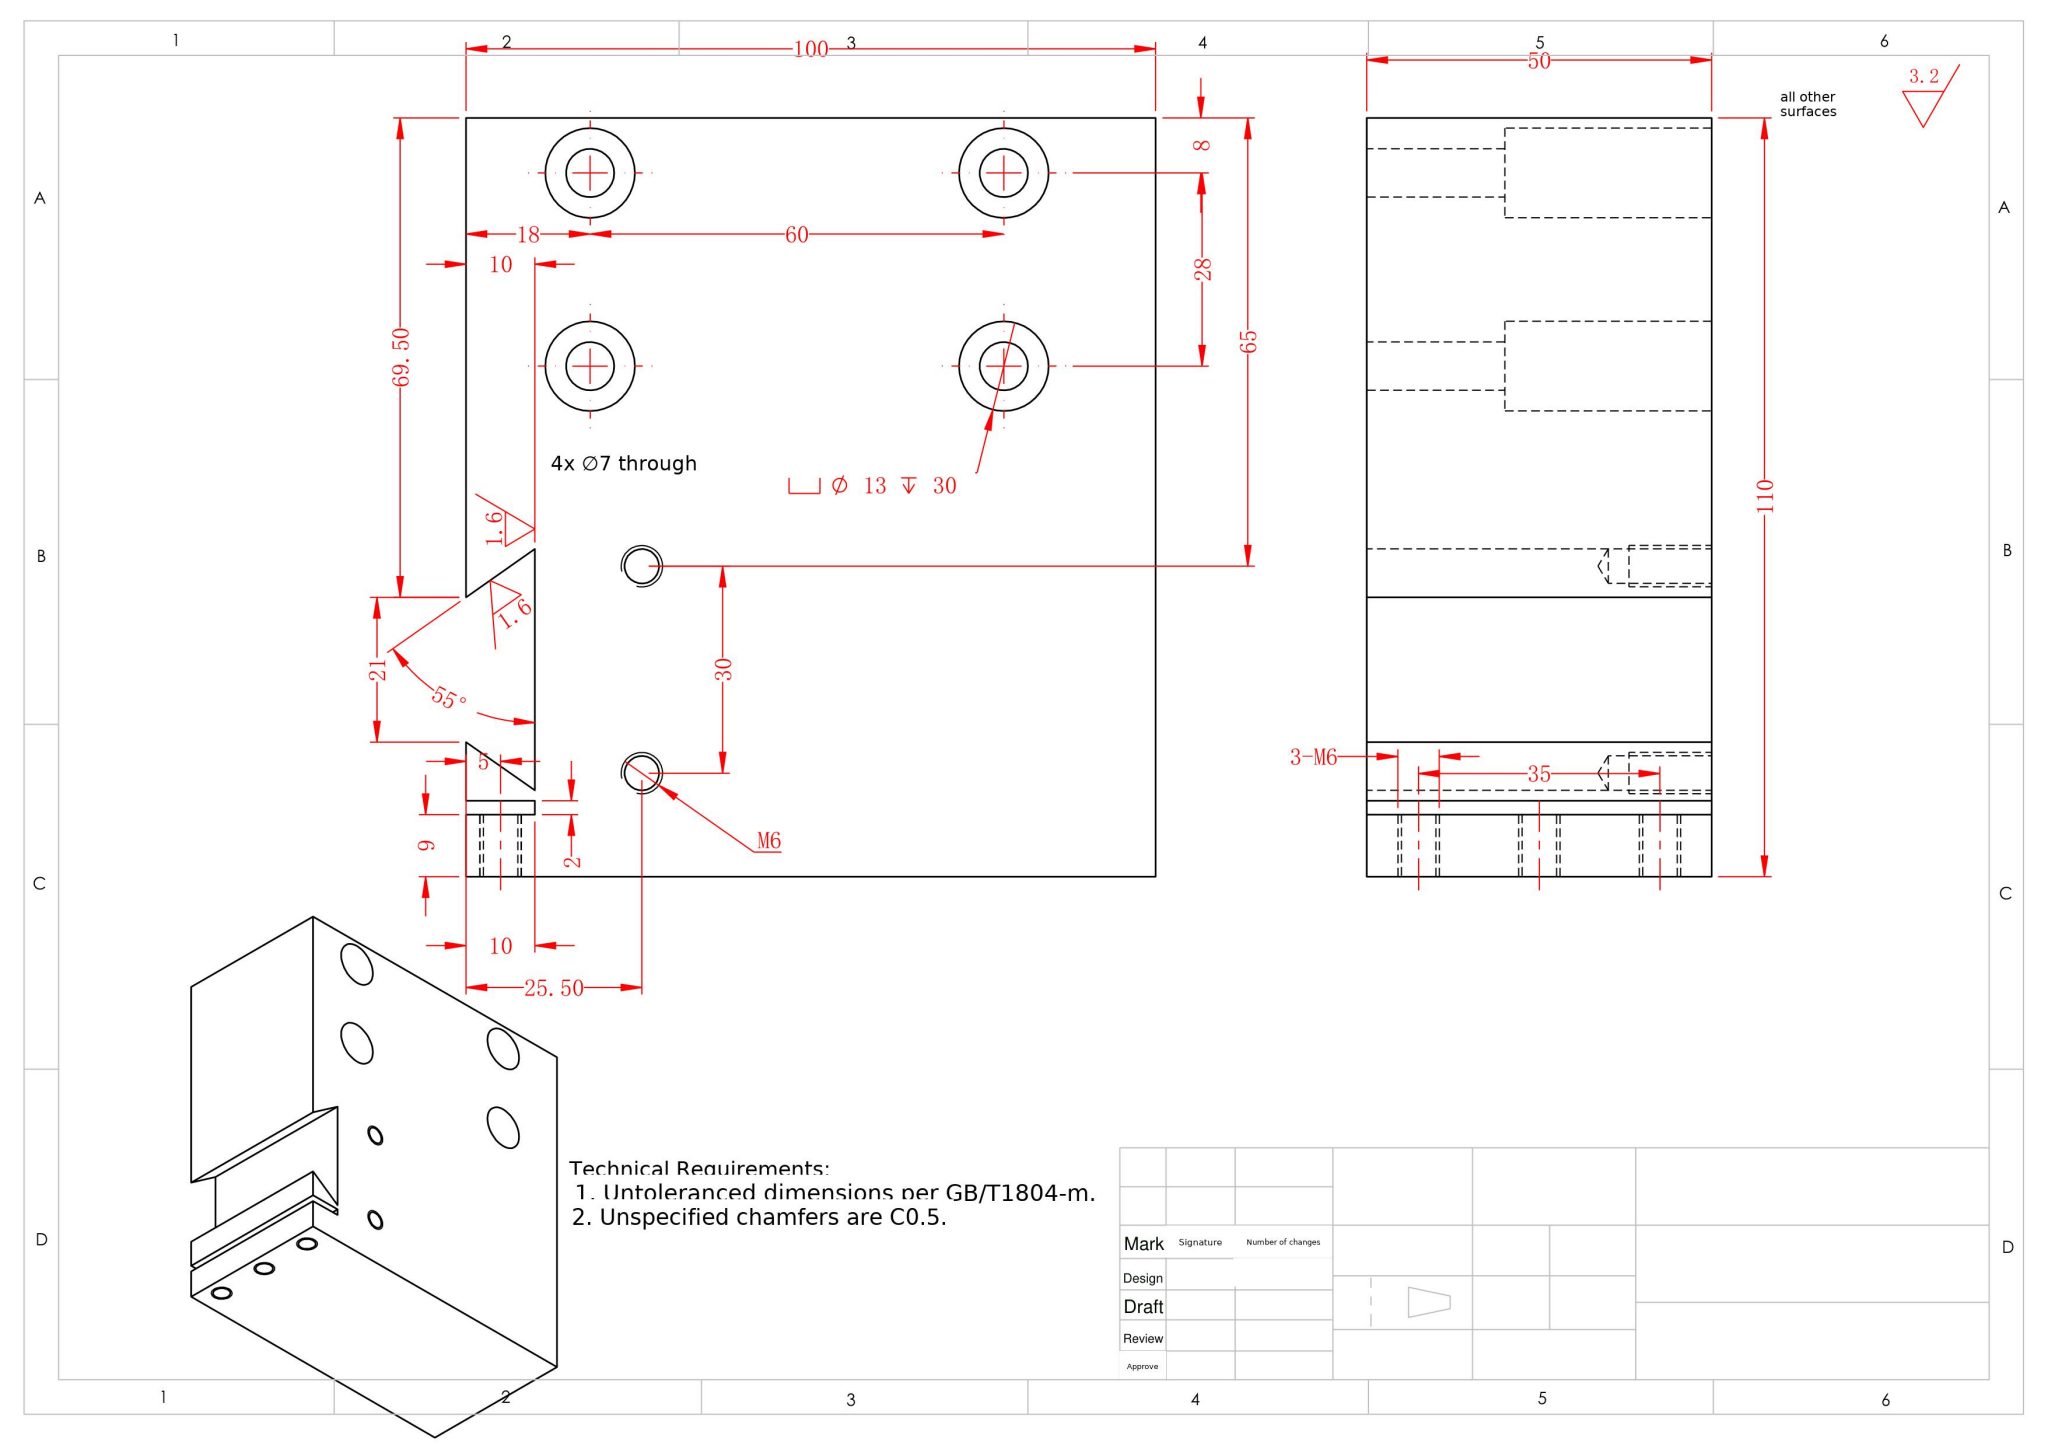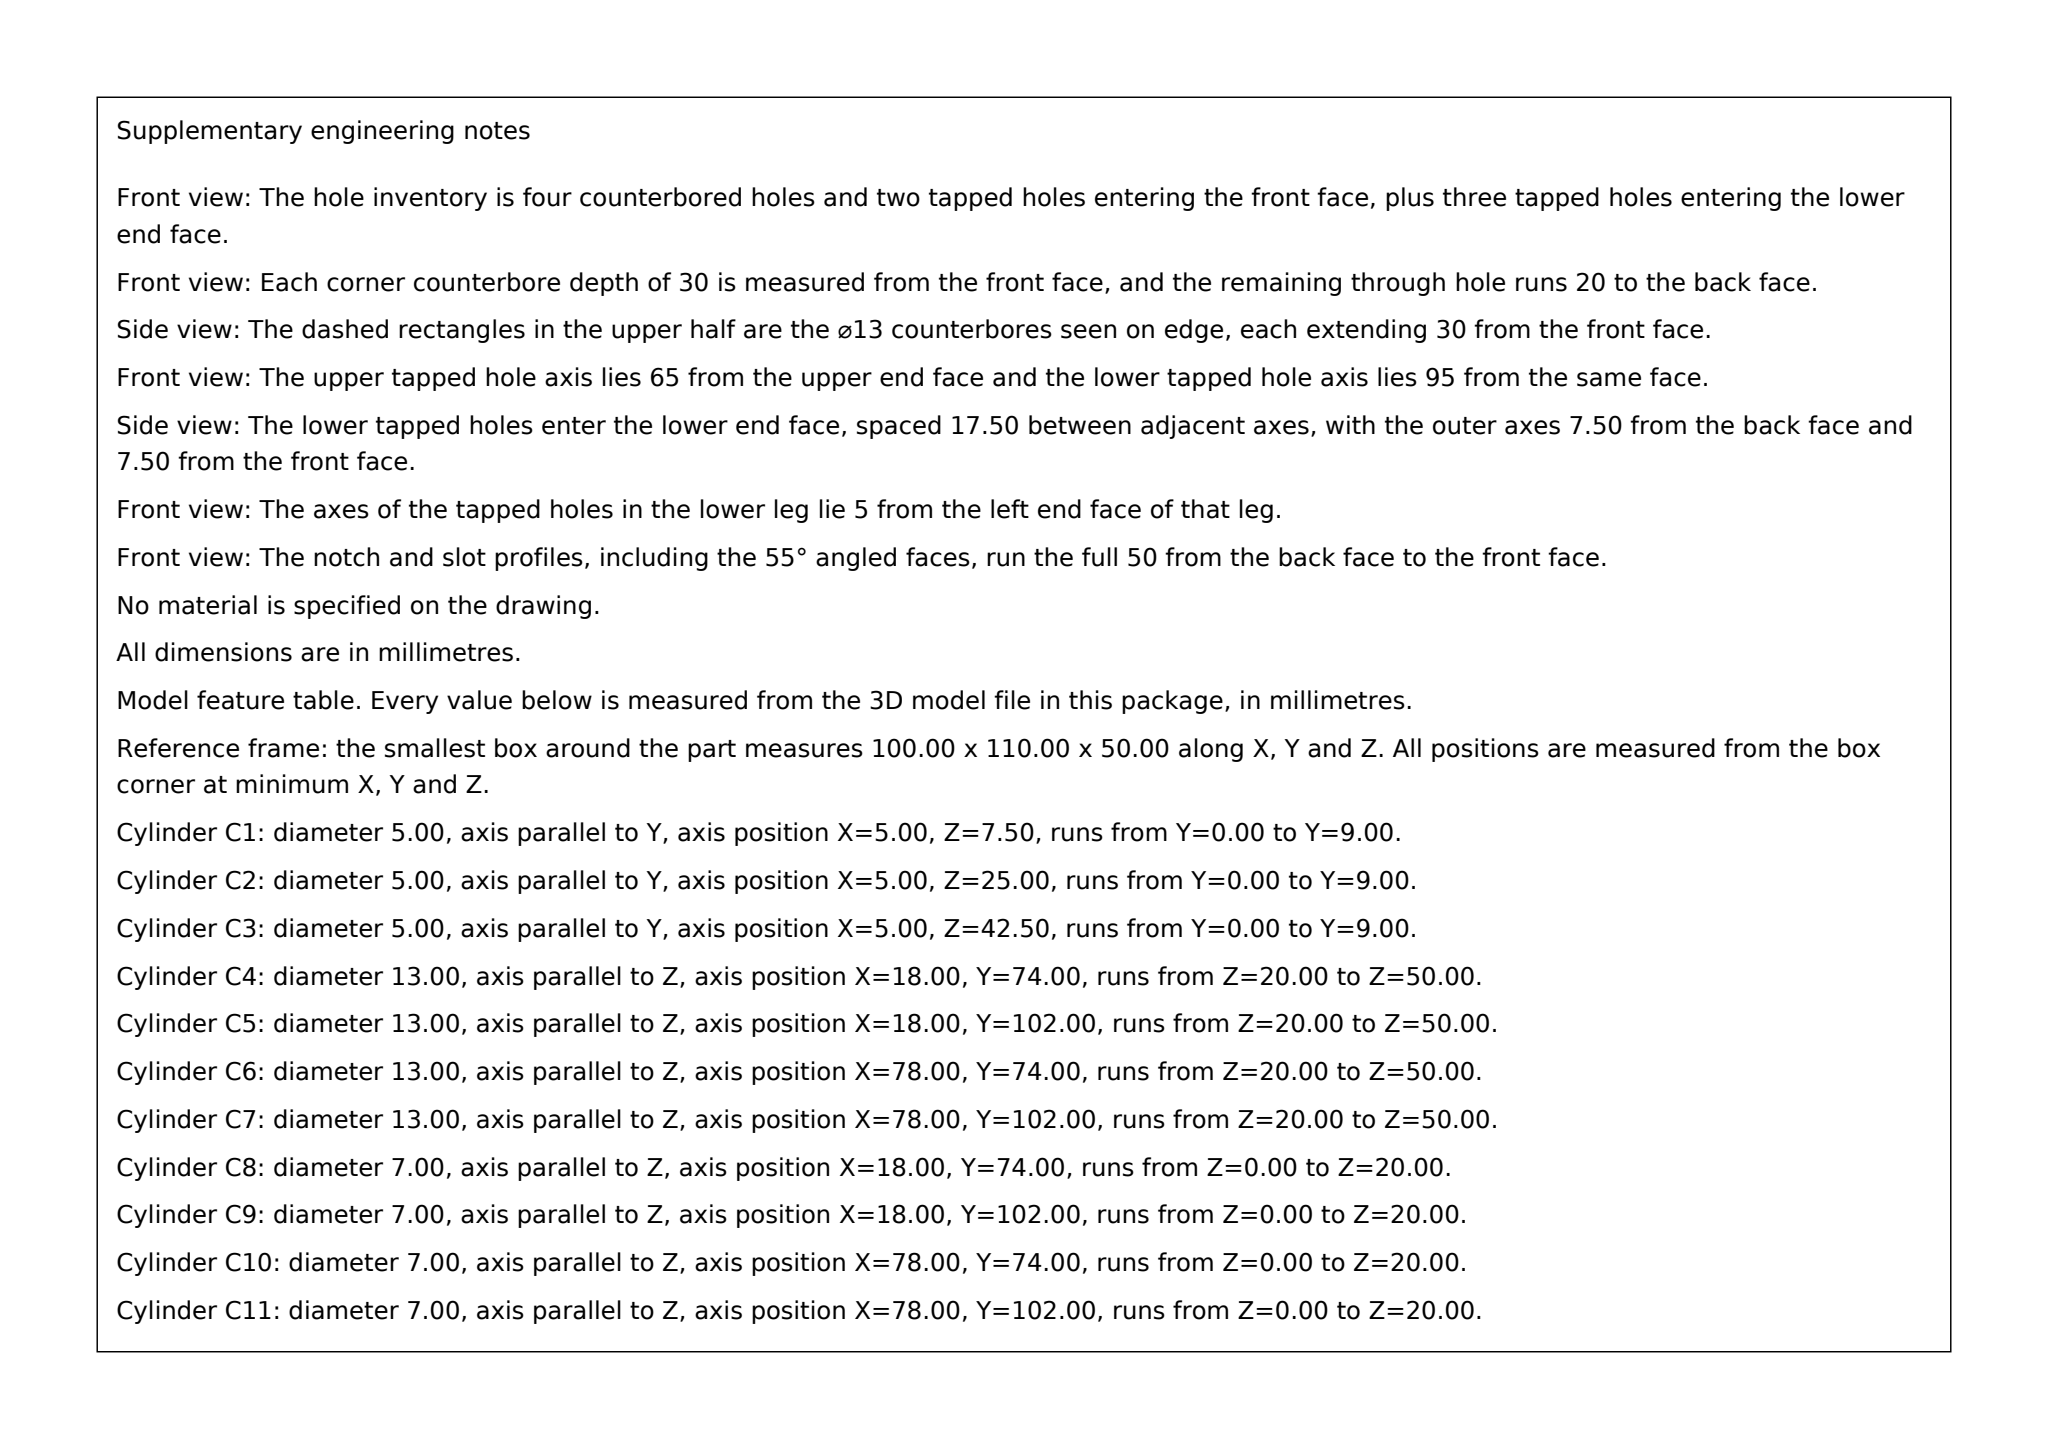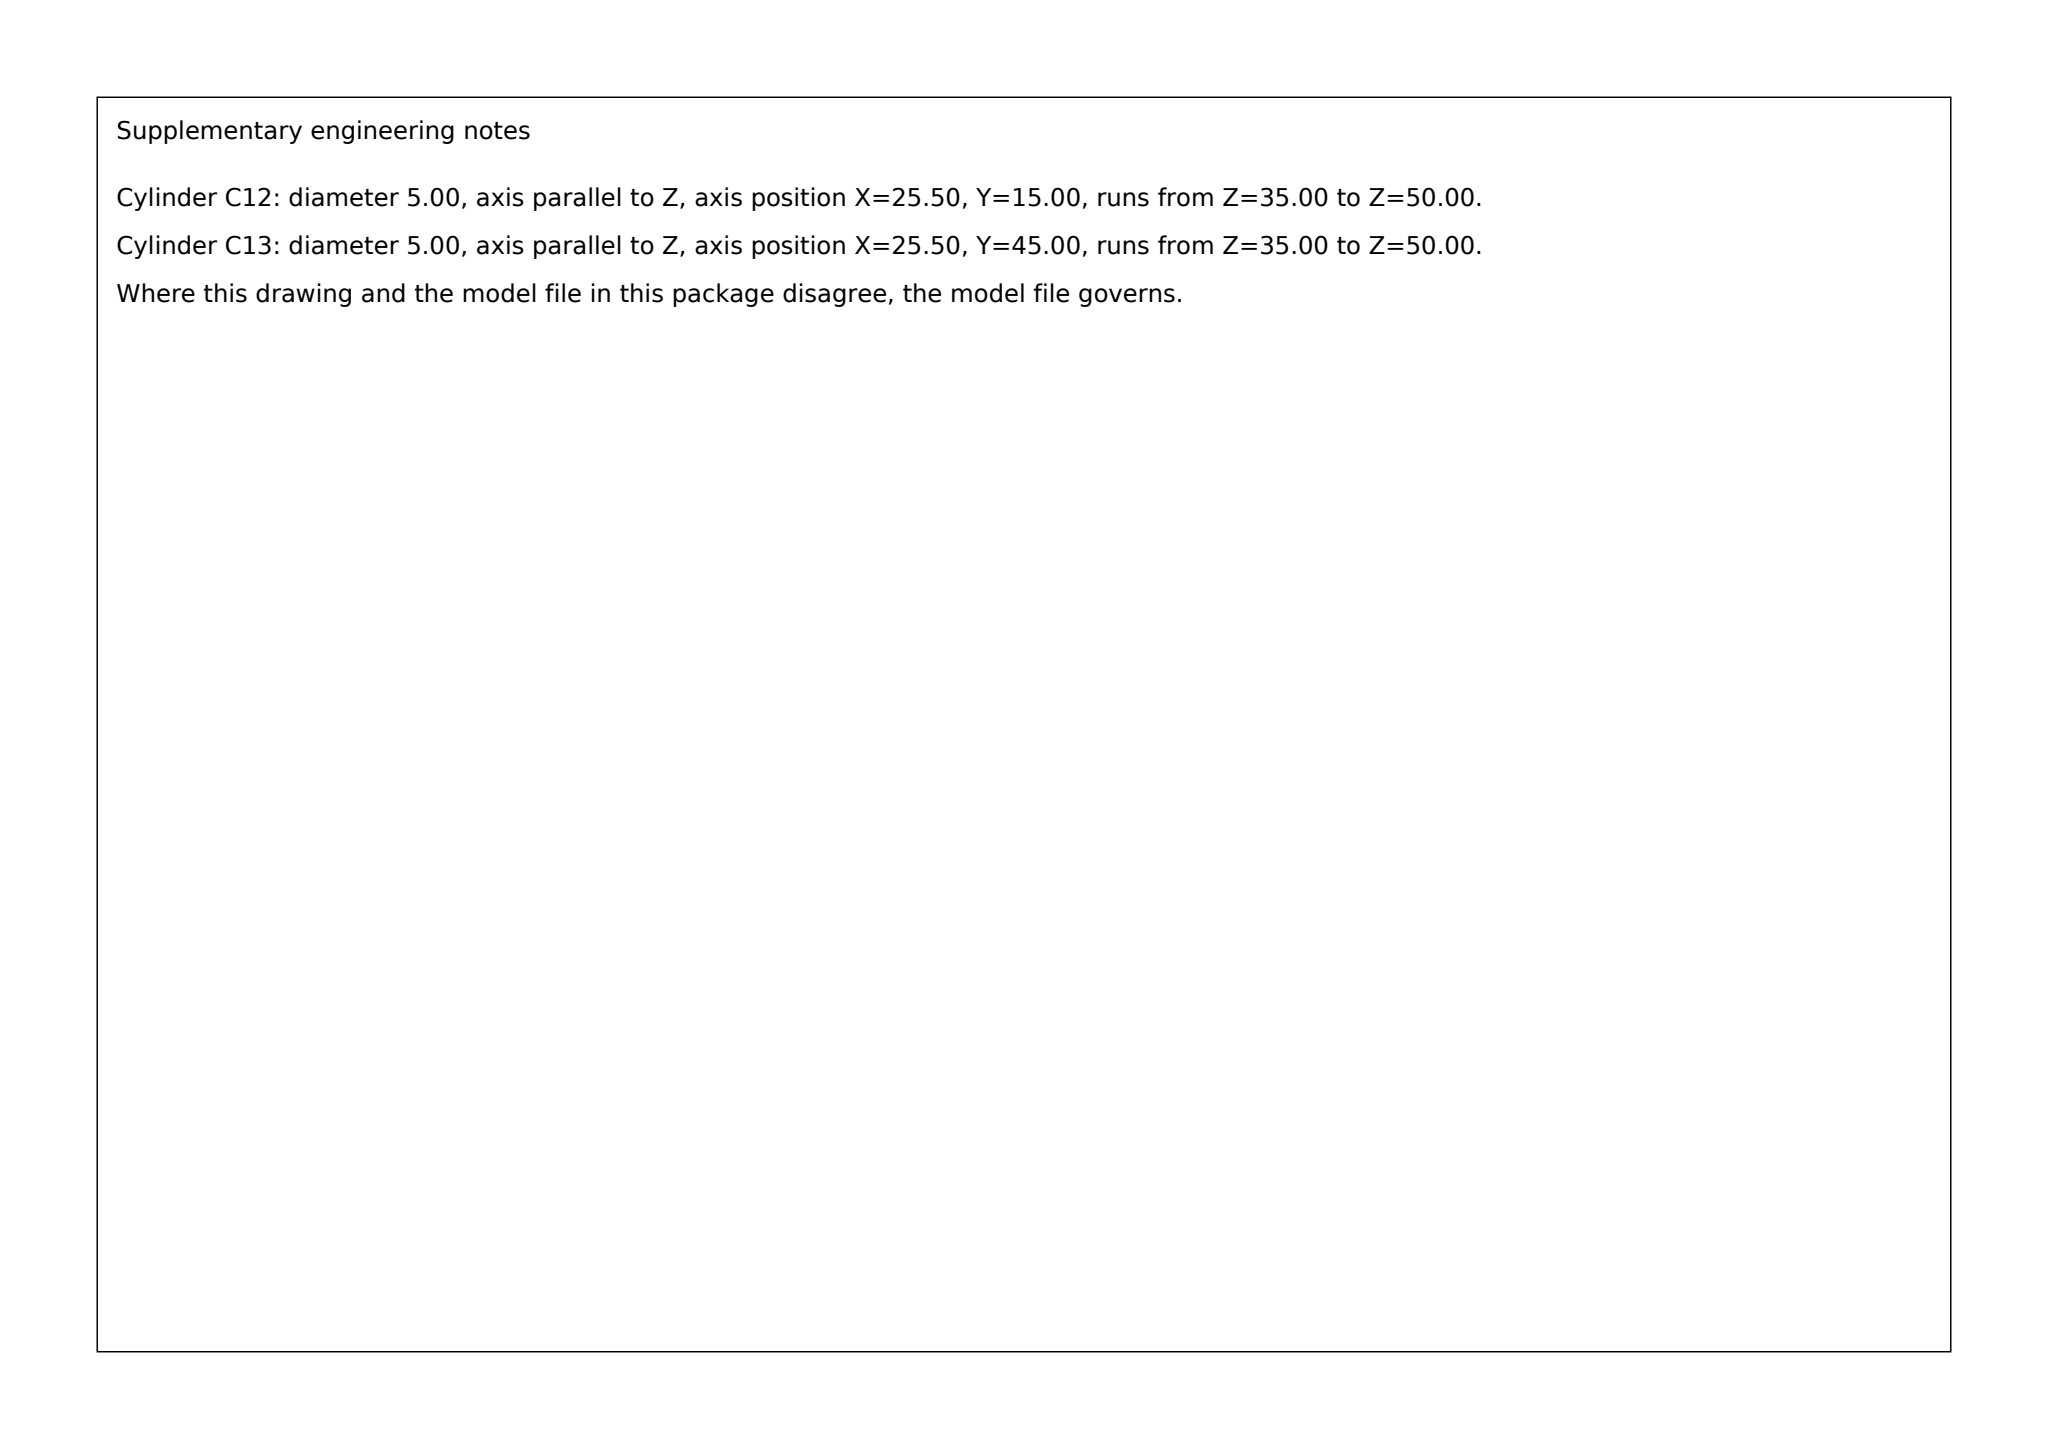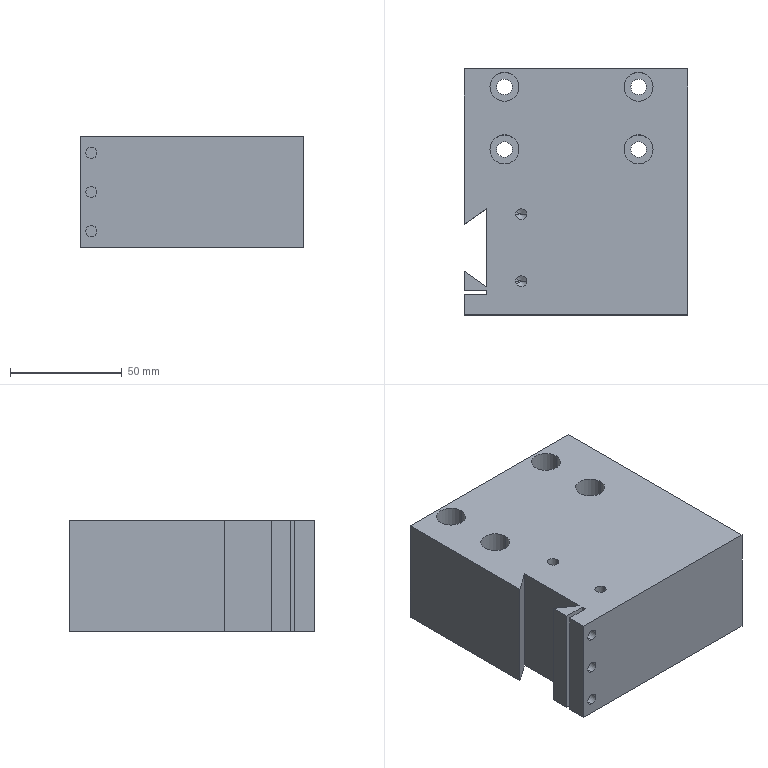Part | SolidWorks | mm | 1 solid | 48 faces | box 100 x 110 x 50 mm | volume 514856 mm3 | cylinder 26 | plane 18 | cone 4 | commonest cylinder face diameters 5 x10 13 x8 7 x8
Drawing notes:
3X M6 DP 9 IN FOOT: HOLE CL 5 FROM FOOT FACE (10 THK) | from the solid: Ø5 cyls, axis y, x=5.0, len 9.0; foot faces x=0 and x=10
3X M6 EQ SP 17.50: 7.50, 25, 42.50 FROM FOOT END FACE | from the solid: Ø5 y-axis cyls at z=7.5, 25.0, 42.5; 50 wide face
build123d program:
from build123d import *

# Parameters (mm, degrees)
BOSS_EXTRUDE1_DEPTH                                 = 50
CYLINDRICAL_COUNTERSUNK_HOLE_FOR_M6_HEX_D           = 7
CYLINDRICAL_COUNTERSUNK_HOLE_FOR_M6_HEX_CBORE_D     = 13
CYLINDRICAL_COUNTERSUNK_HOLE_FOR_M6_HEX_CBORE_DEPTH = 30
M6_TAPPED_HOLE1_D                                   = 5
M6_TAPPED_HOLE1_DEPTH                               = 9
M6_TAPPED_HOLE2_D                                   = 5
M6_TAPPED_HOLE2_DEPTH                               = 15
M6_TAPPED_HOLE2_TIP                                 = 1.502


with BuildPart() as part:
    # Sketch1 → Boss-Extrude1 (new body)
    with BuildSketch(Plane.XY):
        Polygon((-50, -14.502), (-40, -7.5), (-40, -42.5), (-50, -35.498), (-50, -44), (-40, -44), (-40, -46), (-50, -46), (-50, -55), (50, -55), (50, 55), (-50, 55), align=None)
    extrude(amount=BOSS_EXTRUDE1_DEPTH)

    # Cylindrical Countersunk Hole for M6 Hex (through all)
    with Locations(Plane.XY.offset(50)):
        with Locations((-32, 47), (28, 47), (28, 19), (-32, 19)):
            CounterBoreHole(CYLINDRICAL_COUNTERSUNK_HOLE_FOR_M6_HEX_D / 2, CYLINDRICAL_COUNTERSUNK_HOLE_FOR_M6_HEX_CBORE_D / 2, CYLINDRICAL_COUNTERSUNK_HOLE_FOR_M6_HEX_CBORE_DEPTH)

    # M6 Tapped Hole1
    with Locations(Plane(origin=(0, -55, 0), x_dir=(-1, 0, 0), z_dir=(0, -1, 0))):
        with Locations((45, -42.5), (45, -25), (45, -7.5)):
            Hole(M6_TAPPED_HOLE1_D / 2, depth=M6_TAPPED_HOLE1_DEPTH)

    # M6 Tapped Hole2
    with Locations(Plane.XY.offset(50)):
        with Locations((-24.5, -10), (-24.5, -40)):
            Hole(M6_TAPPED_HOLE2_D / 2, depth=M6_TAPPED_HOLE2_DEPTH)
            with Locations((0, 0, -(M6_TAPPED_HOLE2_DEPTH + M6_TAPPED_HOLE2_TIP / 2))):  # 118° drill point
                Cone(0, M6_TAPPED_HOLE2_D / 2, M6_TAPPED_HOLE2_TIP, mode=Mode.SUBTRACT)


solid = part.part